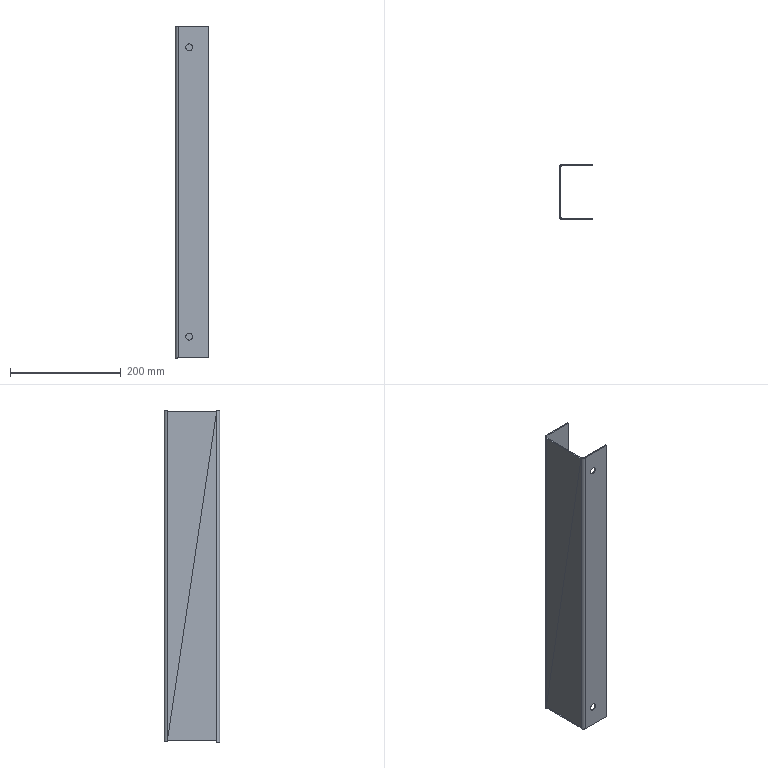Component | SolidWorks | Base-1_BaseLeft-Right-2 | 1 solid | 36 faces | box 60 x 100 x 600 mm | volume 252871 mm3 | plane 24 | cylinder 12 | commonest cylinder face diameters 12.5 x8 7 x2 11 x2
STEP:
#1=COLOUR_RGB('',0.7922,0.8196,0.9333);
#2=FILL_AREA_STYLE_COLOUR('',#1);
#3=FILL_AREA_STYLE('',(#2));
#4=SURFACE_STYLE_FILL_AREA(#3);
#5=SURFACE_SIDE_STYLE('',(#4));
#6=SURFACE_STYLE_USAGE(.BOTH.,#5);
#7=PRESENTATION_STYLE_ASSIGNMENT((#6));
#8=CARTESIAN_POINT('',(-17.788,-8.801,14.723));
#9=VERTEX_POINT('',#8);
#10=CARTESIAN_POINT('',(-18.28,-8.801,14.723));
#11=VERTEX_POINT('',#10);
#12=CARTESIAN_POINT('',(-18.034,-8.801,14.723));
#13=DIRECTION('',(0.,-1.,-0.));
#14=DIRECTION('',(1.,0.,0.));
#15=AXIS2_PLACEMENT_3D('',#12,#13,#14);
#16=CIRCLE('',#15,0.2461);
#17=EDGE_CURVE('',#9,#11,#16,.T.);
#18=ORIENTED_EDGE('',*,*,#17,.F.);
#19=CARTESIAN_POINT('',(-17.788,-8.88,14.723));
#20=VERTEX_POINT('',#19);
#21=CARTESIAN_POINT('',(-17.788,-4.942,14.723));
#22=DIRECTION('',(0.,-1.,-0.));
#23=VECTOR('',#22,39.37);
#24=LINE('',#21,#23);
#25=EDGE_CURVE('',#9,#20,#24,.T.);
#26=ORIENTED_EDGE('',*,*,#25,.T.);
#27=CARTESIAN_POINT('',(-18.28,-8.88,14.723));
#28=VERTEX_POINT('',#27);
#29=CARTESIAN_POINT('',(-18.034,-8.88,14.723));
#30=DIRECTION('',(0.,-1.,-0.));
#31=DIRECTION('',(-1.,-0.,-0.));
#32=AXIS2_PLACEMENT_3D('',#29,#30,#31);
#33=CIRCLE('',#32,0.2461);
#34=EDGE_CURVE('',#20,#28,#33,.T.);
#35=ORIENTED_EDGE('',*,*,#34,.T.);
#36=CARTESIAN_POINT('',(-18.28,-4.942,14.723));
#37=DIRECTION('',(0.,-1.,-0.));
#38=VECTOR('',#37,39.37);
#39=LINE('',#36,#38);
#40=EDGE_CURVE('',#11,#28,#39,.T.);
#41=ORIENTED_EDGE('',*,*,#40,.F.);
#42=EDGE_LOOP('',(#18,#26,#35,#41));
#43=FACE_OUTER_BOUND('',#42,.T.);
#44=CARTESIAN_POINT('',(-18.034,-4.942,14.723));
#45=DIRECTION('',(0.,-1.,-0.));
#46=DIRECTION('',(-1.,-0.,-0.));
#47=AXIS2_PLACEMENT_3D('',#44,#45,#46);
#48=CYLINDRICAL_SURFACE('',#47,0.2461);
#49=ADVANCED_FACE('',(#43),#48,.F.);
#50=CARTESIAN_POINT('',(-17.788,-8.801,-5.867));
#51=VERTEX_POINT('',#50);
#52=CARTESIAN_POINT('',(-18.28,-8.801,-5.867));
#53=VERTEX_POINT('',#52);
#54=CARTESIAN_POINT('',(-18.034,-8.801,-5.867));
#55=DIRECTION('',(0.,-1.,-0.));
#56=DIRECTION('',(1.,0.,0.));
#57=AXIS2_PLACEMENT_3D('',#54,#55,#56);
#58=CIRCLE('',#57,0.2461);
#59=EDGE_CURVE('',#51,#53,#58,.T.);
#60=ORIENTED_EDGE('',*,*,#59,.F.);
#61=CARTESIAN_POINT('',(-17.788,-8.88,-5.867));
#62=VERTEX_POINT('',#61);
#63=CARTESIAN_POINT('',(-17.788,-4.942,-5.867));
#64=DIRECTION('',(0.,-1.,-0.));
#65=VECTOR('',#64,39.37);
#66=LINE('',#63,#65);
#67=EDGE_CURVE('',#51,#62,#66,.T.);
#68=ORIENTED_EDGE('',*,*,#67,.T.);
#69=CARTESIAN_POINT('',(-18.28,-8.88,-5.867));
#70=VERTEX_POINT('',#69);
#71=CARTESIAN_POINT('',(-18.034,-8.88,-5.867));
#72=DIRECTION('',(0.,-1.,-0.));
#73=DIRECTION('',(-1.,-0.,-0.));
#74=AXIS2_PLACEMENT_3D('',#71,#72,#73);
#75=CIRCLE('',#74,0.2461);
#76=EDGE_CURVE('',#62,#70,#75,.T.);
#77=ORIENTED_EDGE('',*,*,#76,.T.);
#78=CARTESIAN_POINT('',(-18.28,-4.942,-5.867));
#79=DIRECTION('',(0.,-1.,-0.));
#80=VECTOR('',#79,39.37);
#81=LINE('',#78,#80);
#82=EDGE_CURVE('',#53,#70,#81,.T.);
#83=ORIENTED_EDGE('',*,*,#82,.F.);
#84=EDGE_LOOP('',(#60,#68,#77,#83));
#85=FACE_OUTER_BOUND('',#84,.T.);
#86=CARTESIAN_POINT('',(-18.034,-4.942,-5.867));
#87=DIRECTION('',(0.,-1.,-0.));
#88=DIRECTION('',(-1.,-0.,-0.));
#89=AXIS2_PLACEMENT_3D('',#86,#87,#88);
#90=CYLINDRICAL_SURFACE('',#89,0.2461);
#91=ADVANCED_FACE('',(#85),#90,.F.);
#92=CARTESIAN_POINT('',(-18.28,-5.021,12.105));
#93=VERTEX_POINT('',#92);
#94=CARTESIAN_POINT('',(-17.788,-5.021,12.105));
#95=VERTEX_POINT('',#94);
#96=CARTESIAN_POINT('',(-18.034,-5.021,12.105));
#97=DIRECTION('',(-0.,1.,0.));
#98=DIRECTION('',(-1.,-0.,-0.));
#99=AXIS2_PLACEMENT_3D('',#96,#97,#98);
#100=CIRCLE('',#99,0.2461);
#101=EDGE_CURVE('',#93,#95,#100,.T.);
#102=ORIENTED_EDGE('',*,*,#101,.F.);
#103=CARTESIAN_POINT('',(-18.28,-4.943,12.105));
#104=VERTEX_POINT('',#103);
#105=CARTESIAN_POINT('',(-18.28,-8.88,12.105));
#106=DIRECTION('',(-0.,1.,0.));
#107=VECTOR('',#106,39.37);
#108=LINE('',#105,#107);
#109=EDGE_CURVE('',#93,#104,#108,.T.);
#110=ORIENTED_EDGE('',*,*,#109,.T.);
#111=CARTESIAN_POINT('',(-17.788,-4.943,12.105));
#112=VERTEX_POINT('',#111);
#113=CARTESIAN_POINT('',(-18.034,-4.943,12.105));
#114=DIRECTION('',(-0.,1.,0.));
#115=DIRECTION('',(1.,0.,0.));
#116=AXIS2_PLACEMENT_3D('',#113,#114,#115);
#117=CIRCLE('',#116,0.2461);
#118=EDGE_CURVE('',#104,#112,#117,.T.);
#119=ORIENTED_EDGE('',*,*,#118,.T.);
#120=CARTESIAN_POINT('',(-17.788,-8.88,12.105));
#121=DIRECTION('',(-0.,1.,0.));
#122=VECTOR('',#121,39.37);
#123=LINE('',#120,#122);
#124=EDGE_CURVE('',#95,#112,#123,.T.);
#125=ORIENTED_EDGE('',*,*,#124,.F.);
#126=EDGE_LOOP('',(#102,#110,#119,#125));
#127=FACE_OUTER_BOUND('',#126,.T.);
#128=CARTESIAN_POINT('',(-18.034,-8.88,12.105));
#129=DIRECTION('',(-0.,1.,0.));
#130=DIRECTION('',(1.,0.,0.));
#131=AXIS2_PLACEMENT_3D('',#128,#129,#130);
#132=CYLINDRICAL_SURFACE('',#131,0.2461);
#133=ADVANCED_FACE('',(#127),#132,.F.);
#134=CARTESIAN_POINT('',(-18.28,-5.021,-3.249));
#135=VERTEX_POINT('',#134);
#136=CARTESIAN_POINT('',(-17.788,-5.021,-3.249));
#137=VERTEX_POINT('',#136);
#138=CARTESIAN_POINT('',(-18.034,-5.021,-3.249));
#139=DIRECTION('',(-0.,1.,0.));
#140=DIRECTION('',(-1.,-0.,-0.));
#141=AXIS2_PLACEMENT_3D('',#138,#139,#140);
#142=CIRCLE('',#141,0.2461);
#143=EDGE_CURVE('',#135,#137,#142,.T.);
#144=ORIENTED_EDGE('',*,*,#143,.F.);
#145=CARTESIAN_POINT('',(-18.28,-4.943,-3.249));
#146=VERTEX_POINT('',#145);
#147=CARTESIAN_POINT('',(-18.28,-8.88,-3.249));
#148=DIRECTION('',(-0.,1.,0.));
#149=VECTOR('',#148,39.37);
#150=LINE('',#147,#149);
#151=EDGE_CURVE('',#135,#146,#150,.T.);
#152=ORIENTED_EDGE('',*,*,#151,.T.);
#153=CARTESIAN_POINT('',(-17.788,-4.943,-3.249));
#154=VERTEX_POINT('',#153);
#155=CARTESIAN_POINT('',(-18.034,-4.943,-3.249));
#156=DIRECTION('',(-0.,1.,0.));
#157=DIRECTION('',(1.,0.,0.));
#158=AXIS2_PLACEMENT_3D('',#155,#156,#157);
#159=CIRCLE('',#158,0.2461);
#160=EDGE_CURVE('',#146,#154,#159,.T.);
#161=ORIENTED_EDGE('',*,*,#160,.T.);
#162=CARTESIAN_POINT('',(-17.788,-8.88,-3.249));
#163=DIRECTION('',(-0.,1.,0.));
#164=VECTOR('',#163,39.37);
#165=LINE('',#162,#164);
#166=EDGE_CURVE('',#137,#154,#165,.T.);
#167=ORIENTED_EDGE('',*,*,#166,.F.);
#168=EDGE_LOOP('',(#144,#152,#161,#167));
#169=FACE_OUTER_BOUND('',#168,.T.);
#170=CARTESIAN_POINT('',(-18.034,-8.88,-3.249));
#171=DIRECTION('',(-0.,1.,0.));
#172=DIRECTION('',(1.,0.,0.));
#173=AXIS2_PLACEMENT_3D('',#170,#171,#172);
#174=CYLINDRICAL_SURFACE('',#173,0.2461);
#175=ADVANCED_FACE('',(#169),#174,.F.);
#176=CARTESIAN_POINT('',(-18.939,-8.663,16.239));
#177=VERTEX_POINT('',#176);
#178=CARTESIAN_POINT('',(-18.939,-8.663,16.239));
#179=VERTEX_POINT('',#178);
#180=CARTESIAN_POINT('',(-18.939,-8.88,16.239));
#181=DIRECTION('',(-0.,1.,0.));
#182=VECTOR('',#181,39.37);
#183=LINE('',#180,#182);
#184=EDGE_CURVE('',#177,#179,#183,.T.);
#185=ORIENTED_EDGE('',*,*,#184,.T.);
#186=CARTESIAN_POINT('',(-19.018,-8.663,16.239));
#187=VERTEX_POINT('',#186);
#188=CARTESIAN_POINT('',(-18.802,-8.663,16.239));
#189=DIRECTION('',(-1.,-0.,-0.));
#190=VECTOR('',#189,39.37);
#191=LINE('',#188,#190);
#192=EDGE_CURVE('',#179,#187,#191,.T.);
#193=ORIENTED_EDGE('',*,*,#192,.T.);
#194=CARTESIAN_POINT('',(-19.018,-8.663,16.239));
#195=DIRECTION('',(1.,0.,0.));
#196=VECTOR('',#195,39.37);
#197=LINE('',#194,#196);
#198=EDGE_CURVE('',#187,#177,#197,.T.);
#199=ORIENTED_EDGE('',*,*,#198,.T.);
#200=EDGE_LOOP('',(#185,#193,#199));
#201=FACE_OUTER_BOUND('',#200,.T.);
#202=CARTESIAN_POINT('',(-18.802,-8.801,16.239));
#203=DIRECTION('',(-0.,-0.,1.));
#204=DIRECTION('',(1.,0.,0.));
#205=AXIS2_PLACEMENT_3D('',#202,#203,#204);
#206=PLANE('',#205);
#207=ADVANCED_FACE('',(#201),#206,.T.);
#208=CARTESIAN_POINT('',(-18.939,-5.159,-7.383));
#209=VERTEX_POINT('',#208);
#210=CARTESIAN_POINT('',(-18.802,-5.021,-7.383));
#211=VERTEX_POINT('',#210);
#212=CARTESIAN_POINT('',(-18.802,-5.159,-7.383));
#213=DIRECTION('',(0.,0.,-1.));
#214=DIRECTION('',(-0.,1.,0.));
#215=AXIS2_PLACEMENT_3D('',#212,#213,#214);
#216=CIRCLE('',#215,0.1378);
#217=EDGE_CURVE('',#209,#211,#216,.T.);
#218=ORIENTED_EDGE('',*,*,#217,.F.);
#219=CARTESIAN_POINT('',(-19.018,-5.159,-7.383));
#220=VERTEX_POINT('',#219);
#221=CARTESIAN_POINT('',(-19.018,-5.159,-7.383));
#222=DIRECTION('',(-1.,-0.,-0.));
#223=VECTOR('',#222,39.37);
#224=LINE('',#221,#223);
#225=EDGE_CURVE('',#209,#220,#224,.T.);
#226=ORIENTED_EDGE('',*,*,#225,.T.);
#227=CARTESIAN_POINT('',(-18.802,-4.943,-7.383));
#228=VERTEX_POINT('',#227);
#229=CARTESIAN_POINT('',(-18.802,-5.159,-7.383));
#230=DIRECTION('',(0.,0.,-1.));
#231=DIRECTION('',(1.,0.,0.));
#232=AXIS2_PLACEMENT_3D('',#229,#230,#231);
#233=CIRCLE('',#232,0.2165);
#234=EDGE_CURVE('',#220,#228,#233,.T.);
#235=ORIENTED_EDGE('',*,*,#234,.T.);
#236=CARTESIAN_POINT('',(-18.802,-5.021,-7.383));
#237=DIRECTION('',(-0.,1.,0.));
#238=VECTOR('',#237,39.37);
#239=LINE('',#236,#238);
#240=EDGE_CURVE('',#211,#228,#239,.T.);
#241=ORIENTED_EDGE('',*,*,#240,.F.);
#242=EDGE_LOOP('',(#218,#226,#235,#241));
#243=FACE_OUTER_BOUND('',#242,.T.);
#244=CARTESIAN_POINT('',(-19.018,-5.159,-7.383));
#245=DIRECTION('',(0.,0.,-1.));
#246=DIRECTION('',(-1.,-0.,-0.));
#247=AXIS2_PLACEMENT_3D('',#244,#245,#246);
#248=PLANE('',#247);
#249=ADVANCED_FACE('',(#243),#248,.T.);
#250=CARTESIAN_POINT('',(-18.939,-8.663,-7.383));
#251=VERTEX_POINT('',#250);
#252=CARTESIAN_POINT('',(-19.018,-8.663,-7.383));
#253=VERTEX_POINT('',#252);
#254=CARTESIAN_POINT('',(-18.939,-8.663,-7.383));
#255=DIRECTION('',(-1.,-0.,-0.));
#256=VECTOR('',#255,39.37);
#257=LINE('',#254,#256);
#258=EDGE_CURVE('',#251,#253,#257,.T.);
#259=ORIENTED_EDGE('',*,*,#258,.T.);
#260=CARTESIAN_POINT('',(-18.939,-8.663,-7.383));
#261=VERTEX_POINT('',#260);
#262=CARTESIAN_POINT('',(-18.802,-8.663,-7.383));
#263=DIRECTION('',(1.,0.,0.));
#264=VECTOR('',#263,39.37);
#265=LINE('',#262,#264);
#266=EDGE_CURVE('',#253,#261,#265,.T.);
#267=ORIENTED_EDGE('',*,*,#266,.T.);
#268=CARTESIAN_POINT('',(-18.939,-8.88,-7.383));
#269=DIRECTION('',(-0.,1.,0.));
#270=VECTOR('',#269,39.37);
#271=LINE('',#268,#270);
#272=EDGE_CURVE('',#251,#261,#271,.T.);
#273=ORIENTED_EDGE('',*,*,#272,.F.);
#274=EDGE_LOOP('',(#259,#267,#273));
#275=FACE_OUTER_BOUND('',#274,.T.);
#276=CARTESIAN_POINT('',(-18.802,-5.021,-7.383));
#277=DIRECTION('',(0.,0.,-1.));
#278=DIRECTION('',(-1.,-0.,-0.));
#279=AXIS2_PLACEMENT_3D('',#276,#277,#278);
#280=PLANE('',#279);
#281=ADVANCED_FACE('',(#275),#280,.T.);
#282=CARTESIAN_POINT('',(-19.018,-5.159,16.239));
#283=VERTEX_POINT('',#282);
#284=CARTESIAN_POINT('',(-18.802,-4.943,16.239));
#285=VERTEX_POINT('',#284);
#286=CARTESIAN_POINT('',(-18.802,-5.159,16.239));
#287=DIRECTION('',(0.,0.,-1.));
#288=DIRECTION('',(1.,0.,0.));
#289=AXIS2_PLACEMENT_3D('',#286,#287,#288);
#290=CIRCLE('',#289,0.2165);
#291=EDGE_CURVE('',#283,#285,#290,.T.);
#292=ORIENTED_EDGE('',*,*,#291,.F.);
#293=CARTESIAN_POINT('',(-18.939,-5.159,16.239));
#294=VERTEX_POINT('',#293);
#295=CARTESIAN_POINT('',(-18.802,-5.159,16.239));
#296=DIRECTION('',(1.,0.,0.));
#297=VECTOR('',#296,39.37);
#298=LINE('',#295,#297);
#299=EDGE_CURVE('',#283,#294,#298,.T.);
#300=ORIENTED_EDGE('',*,*,#299,.T.);
#301=CARTESIAN_POINT('',(-18.802,-5.021,16.239));
#302=VERTEX_POINT('',#301);
#303=CARTESIAN_POINT('',(-18.802,-5.159,16.239));
#304=DIRECTION('',(0.,0.,-1.));
#305=DIRECTION('',(-0.,1.,0.));
#306=AXIS2_PLACEMENT_3D('',#303,#304,#305);
#307=CIRCLE('',#306,0.1378);
#308=EDGE_CURVE('',#294,#302,#307,.T.);
#309=ORIENTED_EDGE('',*,*,#308,.T.);
#310=CARTESIAN_POINT('',(-18.802,-4.943,16.239));
#311=DIRECTION('',(0.,-1.,-0.));
#312=VECTOR('',#311,39.37);
#313=LINE('',#310,#312);
#314=EDGE_CURVE('',#285,#302,#313,.T.);
#315=ORIENTED_EDGE('',*,*,#314,.F.);
#316=EDGE_LOOP('',(#292,#300,#309,#315));
#317=FACE_OUTER_BOUND('',#316,.T.);
#318=CARTESIAN_POINT('',(-18.802,-4.943,16.239));
#319=DIRECTION('',(-0.,-0.,1.));
#320=DIRECTION('',(1.,0.,0.));
#321=AXIS2_PLACEMENT_3D('',#318,#319,#320);
#322=PLANE('',#321);
#323=ADVANCED_FACE('',(#317),#322,.T.);
#324=ORIENTED_EDGE('',*,*,#308,.F.);
#325=CARTESIAN_POINT('',(-18.939,-5.159,16.16));
#326=VERTEX_POINT('',#325);
#327=CARTESIAN_POINT('',(-18.939,-5.159,-7.383));
#328=DIRECTION('',(0.,0.,-1.));
#329=VECTOR('',#328,39.37);
#330=LINE('',#327,#329);
#331=EDGE_CURVE('',#294,#326,#330,.T.);
#332=ORIENTED_EDGE('',*,*,#331,.T.);
#333=CARTESIAN_POINT('',(-18.939,-5.159,-7.304));
#334=VERTEX_POINT('',#333);
#335=CARTESIAN_POINT('',(-18.939,-5.159,-7.383));
#336=DIRECTION('',(-0.,-0.,1.));
#337=VECTOR('',#336,39.37);
#338=LINE('',#335,#337);
#339=EDGE_CURVE('',#334,#326,#338,.T.);
#340=ORIENTED_EDGE('',*,*,#339,.F.);
#341=CARTESIAN_POINT('',(-18.939,-5.159,-7.383));
#342=DIRECTION('',(0.,0.,-1.));
#343=VECTOR('',#342,39.37);
#344=LINE('',#341,#343);
#345=EDGE_CURVE('',#334,#209,#344,.T.);
#346=ORIENTED_EDGE('',*,*,#345,.T.);
#347=ORIENTED_EDGE('',*,*,#217,.T.);
#348=CARTESIAN_POINT('',(-18.802,-5.021,-7.383));
#349=DIRECTION('',(-0.,-0.,1.));
#350=VECTOR('',#349,39.37);
#351=LINE('',#348,#350);
#352=EDGE_CURVE('',#211,#302,#351,.T.);
#353=ORIENTED_EDGE('',*,*,#352,.T.);
#354=EDGE_LOOP('',(#324,#332,#340,#346,#347,#353));
#355=FACE_OUTER_BOUND('',#354,.T.);
#356=CARTESIAN_POINT('',(-18.802,-5.159,-7.383));
#357=DIRECTION('',(-0.,-0.,1.));
#358=DIRECTION('',(1.,0.,0.));
#359=AXIS2_PLACEMENT_3D('',#356,#357,#358);
#360=CYLINDRICAL_SURFACE('',#359,0.1378);
#361=ADVANCED_FACE('',(#355),#360,.F.);
#362=CARTESIAN_POINT('',(-18.939,-8.663,16.16));
#363=VERTEX_POINT('',#362);
#364=CARTESIAN_POINT('',(-18.939,-8.88,16.16));
#365=DIRECTION('',(0.,-1.,-0.));
#366=VECTOR('',#365,39.37);
#367=LINE('',#364,#366);
#368=EDGE_CURVE('',#326,#363,#367,.T.);
#369=ORIENTED_EDGE('',*,*,#368,.T.);
#370=CARTESIAN_POINT('',(-18.939,-8.663,-7.383));
#371=DIRECTION('',(-0.,-0.,1.));
#372=VECTOR('',#371,39.37);
#373=LINE('',#370,#372);
#374=EDGE_CURVE('',#363,#179,#373,.T.);
#375=ORIENTED_EDGE('',*,*,#374,.T.);
#376=ORIENTED_EDGE('',*,*,#184,.F.);
#377=CARTESIAN_POINT('',(-18.939,-8.663,-7.383));
#378=DIRECTION('',(-0.,-0.,1.));
#379=VECTOR('',#378,39.37);
#380=LINE('',#377,#379);
#381=EDGE_CURVE('',#251,#177,#380,.T.);
#382=ORIENTED_EDGE('',*,*,#381,.F.);
#383=ORIENTED_EDGE('',*,*,#272,.T.);
#384=CARTESIAN_POINT('',(-18.939,-8.663,-7.304));
#385=VERTEX_POINT('',#384);
#386=CARTESIAN_POINT('',(-18.939,-8.663,-7.383));
#387=DIRECTION('',(-0.,-0.,1.));
#388=VECTOR('',#387,39.37);
#389=LINE('',#386,#388);
#390=EDGE_CURVE('',#261,#385,#389,.T.);
#391=ORIENTED_EDGE('',*,*,#390,.T.);
#392=CARTESIAN_POINT('',(-18.939,-8.88,-7.304));
#393=DIRECTION('',(-0.,1.,0.));
#394=VECTOR('',#393,39.37);
#395=LINE('',#392,#394);
#396=EDGE_CURVE('',#385,#334,#395,.T.);
#397=ORIENTED_EDGE('',*,*,#396,.T.);
#398=ORIENTED_EDGE('',*,*,#339,.T.);
#399=EDGE_LOOP('',(#369,#375,#376,#382,#383,#391,#397,#398));
#400=FACE_OUTER_BOUND('',#399,.T.);
#401=CARTESIAN_POINT('',(-18.939,-8.88,-7.383));
#402=DIRECTION('',(1.,0.,0.));
#403=DIRECTION('',(0.,-1.,-0.));
#404=AXIS2_PLACEMENT_3D('',#401,#402,#403);
#405=PLANE('',#404);
#406=ADVANCED_FACE('',(#400),#405,.T.);
#407=CARTESIAN_POINT('',(-19.018,-8.663,16.16));
#408=VERTEX_POINT('',#407);
#409=CARTESIAN_POINT('',(-19.018,-8.663,16.259));
#410=DIRECTION('',(-0.,-0.,1.));
#411=VECTOR('',#410,39.37);
#412=LINE('',#409,#411);
#413=EDGE_CURVE('',#408,#187,#412,.T.);
#414=ORIENTED_EDGE('',*,*,#413,.F.);
#415=CARTESIAN_POINT('',(-19.018,-5.159,16.16));
#416=VERTEX_POINT('',#415);
#417=CARTESIAN_POINT('',(-19.018,-8.663,16.16));
#418=DIRECTION('',(0.,-1.,-0.));
#419=VECTOR('',#418,39.37);
#420=LINE('',#417,#419);
#421=EDGE_CURVE('',#416,#408,#420,.T.);
#422=ORIENTED_EDGE('',*,*,#421,.F.);
#423=CARTESIAN_POINT('',(-19.018,-5.159,-7.304));
#424=VERTEX_POINT('',#423);
#425=CARTESIAN_POINT('',(-19.018,-5.159,-7.383));
#426=DIRECTION('',(-0.,-0.,1.));
#427=VECTOR('',#426,39.37);
#428=LINE('',#425,#427);
#429=EDGE_CURVE('',#424,#416,#428,.T.);
#430=ORIENTED_EDGE('',*,*,#429,.F.);
#431=CARTESIAN_POINT('',(-19.018,-8.663,-7.304));
#432=VERTEX_POINT('',#431);
#433=CARTESIAN_POINT('',(-19.018,-8.663,-7.304));
#434=DIRECTION('',(-0.,1.,0.));
#435=VECTOR('',#434,39.37);
#436=LINE('',#433,#435);
#437=EDGE_CURVE('',#432,#424,#436,.T.);
#438=ORIENTED_EDGE('',*,*,#437,.F.);
#439=CARTESIAN_POINT('',(-19.018,-8.663,-7.304));
#440=DIRECTION('',(-0.,-0.,1.));
#441=VECTOR('',#440,39.37);
#442=LINE('',#439,#441);
#443=EDGE_CURVE('',#253,#432,#442,.T.);
#444=ORIENTED_EDGE('',*,*,#443,.F.);
#445=CARTESIAN_POINT('',(-19.018,-8.663,-7.383));
#446=DIRECTION('',(-0.,-0.,1.));
#447=VECTOR('',#446,39.37);
#448=LINE('',#445,#447);
#449=EDGE_CURVE('',#253,#187,#448,.T.);
#450=ORIENTED_EDGE('',*,*,#449,.T.);
#451=EDGE_LOOP('',(#414,#422,#430,#438,#444,#450));
#452=FACE_OUTER_BOUND('',#451,.T.);
#453=CARTESIAN_POINT('',(-19.018,-8.88,-7.383));
#454=DIRECTION('',(1.,0.,0.));
#455=DIRECTION('',(0.,-1.,-0.));
#456=AXIS2_PLACEMENT_3D('',#453,#454,#455);
#457=PLANE('',#456);
#458=ADVANCED_FACE('',(#452),#457,.F.);
#459=CARTESIAN_POINT('',(-18.802,-8.88,-7.383));
#460=VERTEX_POINT('',#459);
#461=CARTESIAN_POINT('',(-18.802,-8.801,-7.383));
#462=VERTEX_POINT('',#461);
#463=CARTESIAN_POINT('',(-18.802,-8.88,-7.383));
#464=DIRECTION('',(-0.,1.,0.));
#465=VECTOR('',#464,39.37);
#466=LINE('',#463,#465);
#467=EDGE_CURVE('',#460,#462,#466,.T.);
#468=ORIENTED_EDGE('',*,*,#467,.F.);
#469=CARTESIAN_POINT('',(-18.802,-8.663,-7.383));
#470=DIRECTION('',(0.,0.,-1.));
#471=DIRECTION('',(1.,0.,0.));
#472=AXIS2_PLACEMENT_3D('',#469,#470,#471);
#473=CIRCLE('',#472,0.2165);
#474=EDGE_CURVE('',#460,#253,#473,.T.);
#475=ORIENTED_EDGE('',*,*,#474,.T.);
#476=ORIENTED_EDGE('',*,*,#258,.F.);
#477=CARTESIAN_POINT('',(-18.802,-8.663,-7.383));
#478=DIRECTION('',(0.,0.,-1.));
#479=DIRECTION('',(-0.,1.,0.));
#480=AXIS2_PLACEMENT_3D('',#477,#478,#479);
#481=CIRCLE('',#480,0.1378);
#482=EDGE_CURVE('',#462,#251,#481,.T.);
#483=ORIENTED_EDGE('',*,*,#482,.F.);
#484=EDGE_LOOP('',(#468,#475,#476,#483));
#485=FACE_OUTER_BOUND('',#484,.T.);
#486=CARTESIAN_POINT('',(-18.802,-8.88,-7.383));
#487=DIRECTION('',(0.,0.,-1.));
#488=DIRECTION('',(-1.,-0.,-0.));
#489=AXIS2_PLACEMENT_3D('',#486,#487,#488);
#490=PLANE('',#489);
#491=ADVANCED_FACE('',(#485),#490,.T.);
#492=CARTESIAN_POINT('',(-16.656,-8.88,-7.383));
#493=VERTEX_POINT('',#492);
#494=CARTESIAN_POINT('',(-16.656,-8.88,-7.383));
#495=DIRECTION('',(-1.,-0.,-0.));
#496=VECTOR('',#495,39.37);
#497=LINE('',#494,#496);
#498=EDGE_CURVE('',#493,#460,#497,.T.);
#499=ORIENTED_EDGE('',*,*,#498,.T.);
#500=ORIENTED_EDGE('',*,*,#467,.T.);
#501=CARTESIAN_POINT('',(-16.656,-8.801,-7.383));
#502=VERTEX_POINT('',#501);
#503=CARTESIAN_POINT('',(-16.656,-8.801,-7.383));
#504=DIRECTION('',(-1.,-0.,-0.));
#505=VECTOR('',#504,39.37);
#506=LINE('',#503,#505);
#507=EDGE_CURVE('',#502,#462,#506,.T.);
#508=ORIENTED_EDGE('',*,*,#507,.F.);
#509=CARTESIAN_POINT('',(-16.656,-8.88,-7.383));
#510=DIRECTION('',(-0.,1.,0.));
#511=VECTOR('',#510,39.37);
#512=LINE('',#509,#511);
#513=EDGE_CURVE('',#493,#502,#512,.T.);
#514=ORIENTED_EDGE('',*,*,#513,.F.);
#515=EDGE_LOOP('',(#499,#500,#508,#514));
#516=FACE_OUTER_BOUND('',#515,.T.);
#517=CARTESIAN_POINT('',(-18.939,-8.663,-7.383));
#518=DIRECTION('',(0.,0.,-1.));
#519=DIRECTION('',(-1.,-0.,-0.));
#520=AXIS2_PLACEMENT_3D('',#517,#518,#519);
#521=PLANE('',#520);
#522=ADVANCED_FACE('',(#516),#521,.T.);
#523=ORIENTED_EDGE('',*,*,#198,.F.);
#524=CARTESIAN_POINT('',(-18.802,-8.88,16.239));
#525=VERTEX_POINT('',#524);
#526=CARTESIAN_POINT('',(-18.802,-8.663,16.239));
#527=DIRECTION('',(0.,0.,-1.));
#528=DIRECTION('',(1.,0.,0.));
#529=AXIS2_PLACEMENT_3D('',#526,#527,#528);
#530=CIRCLE('',#529,0.2165);
#531=EDGE_CURVE('',#525,#187,#530,.T.);
#532=ORIENTED_EDGE('',*,*,#531,.F.);
#533=CARTESIAN_POINT('',(-18.802,-8.801,16.239));
#534=VERTEX_POINT('',#533);
#535=CARTESIAN_POINT('',(-18.802,-8.801,16.239));
#536=DIRECTION('',(0.,-1.,-0.));
#537=VECTOR('',#536,39.37);
#538=LINE('',#535,#537);
#539=EDGE_CURVE('',#534,#525,#538,.T.);
#540=ORIENTED_EDGE('',*,*,#539,.F.);
#541=CARTESIAN_POINT('',(-18.802,-8.663,16.239));
#542=DIRECTION('',(0.,0.,-1.));
#543=DIRECTION('',(-0.,1.,0.));
#544=AXIS2_PLACEMENT_3D('',#541,#542,#543);
#545=CIRCLE('',#544,0.1378);
#546=EDGE_CURVE('',#534,#177,#545,.T.);
#547=ORIENTED_EDGE('',*,*,#546,.T.);
#548=EDGE_LOOP('',(#523,#532,#540,#547));
#549=FACE_OUTER_BOUND('',#548,.T.);
#550=CARTESIAN_POINT('',(-19.018,-8.663,16.239));
#551=DIRECTION('',(-0.,-0.,1.));
#552=DIRECTION('',(1.,0.,0.));
#553=AXIS2_PLACEMENT_3D('',#550,#551,#552);
#554=PLANE('',#553);
#555=ADVANCED_FACE('',(#549),#554,.T.);
#556=CARTESIAN_POINT('',(-16.656,-4.943,16.239));
#557=VERTEX_POINT('',#556);
#558=CARTESIAN_POINT('',(-19.018,-4.943,16.239));
#559=DIRECTION('',(1.,0.,0.));
#560=VECTOR('',#559,39.37);
#561=LINE('',#558,#560);
#562=EDGE_CURVE('',#285,#557,#561,.T.);
#563=ORIENTED_EDGE('',*,*,#562,.F.);
#564=ORIENTED_EDGE('',*,*,#314,.T.);
#565=CARTESIAN_POINT('',(-16.656,-5.021,16.239));
#566=VERTEX_POINT('',#565);
#567=CARTESIAN_POINT('',(-19.018,-5.021,16.239));
#568=DIRECTION('',(1.,0.,0.));
#569=VECTOR('',#568,39.37);
#570=LINE('',#567,#569);
#571=EDGE_CURVE('',#302,#566,#570,.T.);
#572=ORIENTED_EDGE('',*,*,#571,.T.);
#573=CARTESIAN_POINT('',(-16.656,-5.021,16.239));
#574=DIRECTION('',(-0.,1.,0.));
#575=VECTOR('',#574,39.37);
#576=LINE('',#573,#575);
#577=EDGE_CURVE('',#566,#557,#576,.T.);
#578=ORIENTED_EDGE('',*,*,#577,.T.);
#579=EDGE_LOOP('',(#563,#564,#572,#578));
#580=FACE_OUTER_BOUND('',#579,.T.);
#581=CARTESIAN_POINT('',(-18.939,-5.159,16.239));
#582=DIRECTION('',(-0.,-0.,1.));
#583=DIRECTION('',(1.,0.,0.));
#584=AXIS2_PLACEMENT_3D('',#581,#582,#583);
#585=PLANE('',#584);
#586=ADVANCED_FACE('',(#580),#585,.T.);
#587=CARTESIAN_POINT('',(-18.034,-4.943,12.105));
#588=DIRECTION('',(-0.,1.,0.));
#589=DIRECTION('',(1.,0.,0.));
#590=AXIS2_PLACEMENT_3D('',#587,#588,#589);
#591=CIRCLE('',#590,0.2461);
#592=EDGE_CURVE('',#112,#104,#591,.T.);
#593=ORIENTED_EDGE('',*,*,#592,.F.);
#594=ORIENTED_EDGE('',*,*,#118,.F.);
#595=EDGE_LOOP('',(#593,#594));
#596=FACE_BOUND('',#595,.T.);
#597=CARTESIAN_POINT('',(-18.034,-4.943,-3.249));
#598=DIRECTION('',(-0.,1.,0.));
#599=DIRECTION('',(1.,0.,0.));
#600=AXIS2_PLACEMENT_3D('',#597,#598,#599);
#601=CIRCLE('',#600,0.2461);
#602=EDGE_CURVE('',#154,#146,#601,.T.);
#603=ORIENTED_EDGE('',*,*,#602,.F.);
#604=ORIENTED_EDGE('',*,*,#160,.F.);
#605=EDGE_LOOP('',(#603,#604));
#606=FACE_BOUND('',#605,.T.);
#607=ORIENTED_EDGE('',*,*,#562,.T.);
#608=CARTESIAN_POINT('',(-16.656,-4.943,-7.383));
#609=VERTEX_POINT('',#608);
#610=CARTESIAN_POINT('',(-16.656,-4.943,-7.383));
#611=DIRECTION('',(-0.,-0.,1.));
#612=VECTOR('',#611,39.37);
#613=LINE('',#610,#612);
#614=EDGE_CURVE('',#609,#557,#613,.T.);
#615=ORIENTED_EDGE('',*,*,#614,.F.);
#616=CARTESIAN_POINT('',(-19.018,-4.943,-7.383));
#617=DIRECTION('',(1.,0.,0.));
#618=VECTOR('',#617,39.37);
#619=LINE('',#616,#618);
#620=EDGE_CURVE('',#228,#609,#619,.T.);
#621=ORIENTED_EDGE('',*,*,#620,.F.);
#622=CARTESIAN_POINT('',(-18.802,-4.943,-7.383));
#623=DIRECTION('',(-0.,-0.,1.));
#624=VECTOR('',#623,39.37);
#625=LINE('',#622,#624);
#626=EDGE_CURVE('',#228,#285,#625,.T.);
#627=ORIENTED_EDGE('',*,*,#626,.T.);
#628=EDGE_LOOP('',(#607,#615,#621,#627));
#629=FACE_OUTER_BOUND('',#628,.T.);
#630=CARTESIAN_POINT('',(-19.018,-4.943,-7.383));
#631=DIRECTION('',(0.,-1.,-0.));
#632=DIRECTION('',(-1.,-0.,-0.));
#633=AXIS2_PLACEMENT_3D('',#630,#631,#632);
#634=PLANE('',#633);
#635=ADVANCED_FACE('',(#596,#606,#629),#634,.F.);
#636=ORIENTED_EDGE('',*,*,#577,.F.);
#637=CARTESIAN_POINT('',(-16.656,-5.021,-7.383));
#638=VERTEX_POINT('',#637);
#639=CARTESIAN_POINT('',(-16.656,-5.021,-7.383));
#640=DIRECTION('',(-0.,-0.,1.));
#641=VECTOR('',#640,39.37);
#642=LINE('',#639,#641);
#643=EDGE_CURVE('',#638,#566,#642,.T.);
#644=ORIENTED_EDGE('',*,*,#643,.F.);
#645=CARTESIAN_POINT('',(-16.656,-5.021,-7.383));
#646=DIRECTION('',(-0.,1.,0.));
#647=VECTOR('',#646,39.37);
#648=LINE('',#645,#647);
#649=EDGE_CURVE('',#638,#609,#648,.T.);
#650=ORIENTED_EDGE('',*,*,#649,.T.);
#651=ORIENTED_EDGE('',*,*,#614,.T.);
#652=EDGE_LOOP('',(#636,#644,#650,#651));
#653=FACE_OUTER_BOUND('',#652,.T.);
#654=CARTESIAN_POINT('',(-16.656,-5.021,-7.383));
#655=DIRECTION('',(1.,0.,0.));
#656=DIRECTION('',(0.,-1.,-0.));
#657=AXIS2_PLACEMENT_3D('',#654,#655,#656);
#658=PLANE('',#657);
#659=ADVANCED_FACE('',(#653),#658,.T.);
#660=CARTESIAN_POINT('',(-18.034,-5.021,12.105));
#661=DIRECTION('',(-0.,1.,0.));
#662=DIRECTION('',(-1.,-0.,-0.));
#663=AXIS2_PLACEMENT_3D('',#660,#661,#662);
#664=CIRCLE('',#663,0.2461);
#665=EDGE_CURVE('',#95,#93,#664,.T.);
#666=ORIENTED_EDGE('',*,*,#665,.T.);
#667=ORIENTED_EDGE('',*,*,#101,.T.);
#668=EDGE_LOOP('',(#666,#667));
#669=FACE_BOUND('',#668,.T.);
#670=CARTESIAN_POINT('',(-18.034,-5.021,-3.249));
#671=DIRECTION('',(-0.,1.,0.));
#672=DIRECTION('',(-1.,-0.,-0.));
#673=AXIS2_PLACEMENT_3D('',#670,#671,#672);
#674=CIRCLE('',#673,0.2461);
#675=EDGE_CURVE('',#137,#135,#674,.T.);
#676=ORIENTED_EDGE('',*,*,#675,.T.);
#677=ORIENTED_EDGE('',*,*,#143,.T.);
#678=EDGE_LOOP('',(#676,#677));
#679=FACE_BOUND('',#678,.T.);
#680=ORIENTED_EDGE('',*,*,#571,.F.);
#681=ORIENTED_EDGE('',*,*,#352,.F.);
#682=CARTESIAN_POINT('',(-19.018,-5.021,-7.383));
#683=DIRECTION('',(1.,0.,0.));
#684=VECTOR('',#683,39.37);
#685=LINE('',#682,#684);
#686=EDGE_CURVE('',#211,#638,#685,.T.);
#687=ORIENTED_EDGE('',*,*,#686,.T.);
#688=ORIENTED_EDGE('',*,*,#643,.T.);
#689=EDGE_LOOP('',(#680,#681,#687,#688));
#690=FACE_OUTER_BOUND('',#689,.T.);
#691=CARTESIAN_POINT('',(-19.018,-5.021,-7.383));
#692=DIRECTION('',(0.,-1.,-0.));
#693=DIRECTION('',(-1.,-0.,-0.));
#694=AXIS2_PLACEMENT_3D('',#691,#692,#693);
#695=PLANE('',#694);
#696=ADVANCED_FACE('',(#669,#679,#690),#695,.T.);
#697=ORIENTED_EDGE('',*,*,#546,.F.);
#698=CARTESIAN_POINT('',(-18.802,-8.801,-7.383));
#699=DIRECTION('',(-0.,-0.,1.));
#700=VECTOR('',#699,39.37);
#701=LINE('',#698,#700);
#702=EDGE_CURVE('',#462,#534,#701,.T.);
#703=ORIENTED_EDGE('',*,*,#702,.F.);
#704=ORIENTED_EDGE('',*,*,#482,.T.);
#705=ORIENTED_EDGE('',*,*,#381,.T.);
#706=EDGE_LOOP('',(#697,#703,#704,#705));
#707=FACE_OUTER_BOUND('',#706,.T.);
#708=CARTESIAN_POINT('',(-18.802,-8.663,-7.383));
#709=DIRECTION('',(-0.,-0.,1.));
#710=DIRECTION('',(1.,0.,0.));
#711=AXIS2_PLACEMENT_3D('',#708,#709,#710);
#712=CYLINDRICAL_SURFACE('',#711,0.1378);
#713=ADVANCED_FACE('',(#707),#712,.F.);
#714=CARTESIAN_POINT('',(-18.034,-8.801,14.723));
#715=DIRECTION('',(0.,-1.,-0.));
#716=DIRECTION('',(1.,0.,0.));
#717=AXIS2_PLACEMENT_3D('',#714,#715,#716);
#718=CIRCLE('',#717,0.2461);
#719=EDGE_CURVE('',#11,#9,#718,.T.);
#720=ORIENTED_EDGE('',*,*,#719,.T.);
#721=ORIENTED_EDGE('',*,*,#17,.T.);
#722=EDGE_LOOP('',(#720,#721));
#723=FACE_BOUND('',#722,.T.);
#724=CARTESIAN_POINT('',(-18.034,-8.801,-5.867));
#725=DIRECTION('',(0.,-1.,-0.));
#726=DIRECTION('',(1.,0.,0.));
#727=AXIS2_PLACEMENT_3D('',#724,#725,#726);
#728=CIRCLE('',#727,0.2461);
#729=EDGE_CURVE('',#53,#51,#728,.T.);
#730=ORIENTED_EDGE('',*,*,#729,.T.);
#731=ORIENTED_EDGE('',*,*,#59,.T.);
#732=EDGE_LOOP('',(#730,#731));
#733=FACE_BOUND('',#732,.T.);
#734=CARTESIAN_POINT('',(-16.656,-8.801,16.239));
#735=VERTEX_POINT('',#734);
#736=CARTESIAN_POINT('',(-16.656,-8.801,16.239));
#737=DIRECTION('',(-1.,-0.,-0.));
#738=VECTOR('',#737,39.37);
#739=LINE('',#736,#738);
#740=EDGE_CURVE('',#735,#534,#739,.T.);
#741=ORIENTED_EDGE('',*,*,#740,.F.);
#742=CARTESIAN_POINT('',(-16.656,-8.801,-7.383));
#743=DIRECTION('',(-0.,-0.,1.));
#744=VECTOR('',#743,39.37);
#745=LINE('',#742,#744);
#746=EDGE_CURVE('',#502,#735,#745,.T.);
#747=ORIENTED_EDGE('',*,*,#746,.F.);
#748=ORIENTED_EDGE('',*,*,#507,.T.);
#749=ORIENTED_EDGE('',*,*,#702,.T.);
#750=EDGE_LOOP('',(#741,#747,#748,#749));
#751=FACE_OUTER_BOUND('',#750,.T.);
#752=CARTESIAN_POINT('',(-16.656,-8.801,-7.383));
#753=DIRECTION('',(-0.,1.,0.));
#754=DIRECTION('',(1.,0.,0.));
#755=AXIS2_PLACEMENT_3D('',#752,#753,#754);
#756=PLANE('',#755);
#757=ADVANCED_FACE('',(#723,#733,#751),#756,.T.);
#758=CARTESIAN_POINT('',(-16.656,-8.88,16.239));
#759=VERTEX_POINT('',#758);
#760=CARTESIAN_POINT('',(-16.656,-8.88,16.239));
#761=DIRECTION('',(-0.,1.,0.));
#762=VECTOR('',#761,39.37);
#763=LINE('',#760,#762);
#764=EDGE_CURVE('',#759,#735,#763,.T.);
#765=ORIENTED_EDGE('',*,*,#764,.F.);
#766=CARTESIAN_POINT('',(-16.656,-8.88,-7.383));
#767=DIRECTION('',(-0.,-0.,1.));
#768=VECTOR('',#767,39.37);
#769=LINE('',#766,#768);
#770=EDGE_CURVE('',#493,#759,#769,.T.);
#771=ORIENTED_EDGE('',*,*,#770,.F.);
#772=ORIENTED_EDGE('',*,*,#513,.T.);
#773=ORIENTED_EDGE('',*,*,#746,.T.);
#774=EDGE_LOOP('',(#765,#771,#772,#773));
#775=FACE_OUTER_BOUND('',#774,.T.);
#776=CARTESIAN_POINT('',(-16.656,-8.88,-7.383));
#777=DIRECTION('',(1.,0.,0.));
#778=DIRECTION('',(0.,-1.,-0.));
#779=AXIS2_PLACEMENT_3D('',#776,#777,#778);
#780=PLANE('',#779);
#781=ADVANCED_FACE('',(#775),#780,.T.);
#782=CARTESIAN_POINT('',(-18.034,-8.88,14.723));
#783=DIRECTION('',(0.,-1.,-0.));
#784=DIRECTION('',(-1.,-0.,-0.));
#785=AXIS2_PLACEMENT_3D('',#782,#783,#784);
#786=CIRCLE('',#785,0.2461);
#787=EDGE_CURVE('',#28,#20,#786,.T.);
#788=ORIENTED_EDGE('',*,*,#787,.F.);
#789=ORIENTED_EDGE('',*,*,#34,.F.);
#790=EDGE_LOOP('',(#788,#789));
#791=FACE_BOUND('',#790,.T.);
#792=CARTESIAN_POINT('',(-18.034,-8.88,-5.867));
#793=DIRECTION('',(0.,-1.,-0.));
#794=DIRECTION('',(-1.,-0.,-0.));
#795=AXIS2_PLACEMENT_3D('',#792,#793,#794);
#796=CIRCLE('',#795,0.2461);
#797=EDGE_CURVE('',#70,#62,#796,.T.);
#798=ORIENTED_EDGE('',*,*,#797,.F.);
#799=ORIENTED_EDGE('',*,*,#76,.F.);
#800=EDGE_LOOP('',(#798,#799));
#801=FACE_BOUND('',#800,.T.);
#802=CARTESIAN_POINT('',(-16.656,-8.88,16.239));
#803=DIRECTION('',(-1.,-0.,-0.));
#804=VECTOR('',#803,39.37);
#805=LINE('',#802,#804);
#806=EDGE_CURVE('',#759,#525,#805,.T.);
#807=ORIENTED_EDGE('',*,*,#806,.T.);
#808=CARTESIAN_POINT('',(-18.802,-8.88,-7.383));
#809=DIRECTION('',(-0.,-0.,1.));
#810=VECTOR('',#809,39.37);
#811=LINE('',#808,#810);
#812=EDGE_CURVE('',#460,#525,#811,.T.);
#813=ORIENTED_EDGE('',*,*,#812,.F.);
#814=ORIENTED_EDGE('',*,*,#498,.F.);
#815=ORIENTED_EDGE('',*,*,#770,.T.);
#816=EDGE_LOOP('',(#807,#813,#814,#815));
#817=FACE_OUTER_BOUND('',#816,.T.);
#818=CARTESIAN_POINT('',(-16.656,-8.88,-7.383));
#819=DIRECTION('',(-0.,1.,0.));
#820=DIRECTION('',(1.,0.,0.));
#821=AXIS2_PLACEMENT_3D('',#818,#819,#820);
#822=PLANE('',#821);
#823=ADVANCED_FACE('',(#791,#801,#817),#822,.F.);
#824=ORIENTED_EDGE('',*,*,#531,.T.);
#825=ORIENTED_EDGE('',*,*,#449,.F.);
#826=ORIENTED_EDGE('',*,*,#474,.F.);
#827=ORIENTED_EDGE('',*,*,#812,.T.);
#828=EDGE_LOOP('',(#824,#825,#826,#827));
#829=FACE_OUTER_BOUND('',#828,.T.);
#830=CARTESIAN_POINT('',(-18.802,-8.663,-7.383));
#831=DIRECTION('',(-0.,-0.,1.));
#832=DIRECTION('',(1.,0.,0.));
#833=AXIS2_PLACEMENT_3D('',#830,#831,#832);
#834=CYLINDRICAL_SURFACE('',#833,0.2165);
#835=ADVANCED_FACE('',(#829),#834,.T.);
#836=ORIENTED_EDGE('',*,*,#291,.T.);
#837=ORIENTED_EDGE('',*,*,#626,.F.);
#838=ORIENTED_EDGE('',*,*,#234,.F.);
#839=CARTESIAN_POINT('',(-19.018,-5.159,-7.383));
#840=CARTESIAN_POINT('',(-19.018,-5.159,-7.357));
#841=CARTESIAN_POINT('',(-19.018,-5.159,-7.33));
#842=CARTESIAN_POINT('',(-19.018,-5.159,-7.304));
#843=B_SPLINE_CURVE_WITH_KNOTS('',3,(#839,#840,#841,#842),.UNSPECIFIED.,.F.,.F.,(4,4),(0.,0.003333),.UNSPECIFIED.);
#844=EDGE_CURVE('',#220,#424,#843,.T.);
#845=ORIENTED_EDGE('',*,*,#844,.T.);
#846=ORIENTED_EDGE('',*,*,#429,.T.);
#847=CARTESIAN_POINT('',(-19.018,-5.159,16.16));
#848=CARTESIAN_POINT('',(-19.018,-5.159,16.187));
#849=CARTESIAN_POINT('',(-19.018,-5.159,16.213));
#850=CARTESIAN_POINT('',(-19.018,-5.159,16.239));
#851=B_SPLINE_CURVE_WITH_KNOTS('',3,(#847,#848,#849,#850),.UNSPECIFIED.,.F.,.F.,(4,4),(0.9967,1.),.UNSPECIFIED.);
#852=EDGE_CURVE('',#416,#283,#851,.T.);
#853=ORIENTED_EDGE('',*,*,#852,.T.);
#854=EDGE_LOOP('',(#836,#837,#838,#845,#846,#853));
#855=FACE_OUTER_BOUND('',#854,.T.);
#856=CARTESIAN_POINT('',(-18.802,-5.159,-7.383));
#857=DIRECTION('',(-0.,-0.,1.));
#858=DIRECTION('',(1.,0.,0.));
#859=AXIS2_PLACEMENT_3D('',#856,#857,#858);
#860=CYLINDRICAL_SURFACE('',#859,0.2165);
#861=ADVANCED_FACE('',(#855),#860,.T.);
#862=ORIENTED_EDGE('',*,*,#620,.T.);
#863=ORIENTED_EDGE('',*,*,#649,.F.);
#864=ORIENTED_EDGE('',*,*,#686,.F.);
#865=ORIENTED_EDGE('',*,*,#240,.T.);
#866=EDGE_LOOP('',(#862,#863,#864,#865));
#867=FACE_OUTER_BOUND('',#866,.T.);
#868=CARTESIAN_POINT('',(-18.802,-5.159,-7.383));
#869=DIRECTION('',(0.,0.,-1.));
#870=DIRECTION('',(-0.,1.,0.));
#871=AXIS2_PLACEMENT_3D('',#868,#869,#870);
#872=PLANE('',#871);
#873=ADVANCED_FACE('',(#867),#872,.T.);
#874=ORIENTED_EDGE('',*,*,#740,.T.);
#875=ORIENTED_EDGE('',*,*,#539,.T.);
#876=ORIENTED_EDGE('',*,*,#806,.F.);
#877=ORIENTED_EDGE('',*,*,#764,.T.);
#878=EDGE_LOOP('',(#874,#875,#876,#877));
#879=FACE_OUTER_BOUND('',#878,.T.);
#880=CARTESIAN_POINT('',(-18.802,-5.159,16.239));
#881=DIRECTION('',(0.,0.,-1.));
#882=DIRECTION('',(-0.,1.,0.));
#883=AXIS2_PLACEMENT_3D('',#880,#881,#882);
#884=PLANE('',#883);
#885=ADVANCED_FACE('',(#879),#884,.F.);
#886=ORIENTED_EDGE('',*,*,#151,.F.);
#887=ORIENTED_EDGE('',*,*,#675,.F.);
#888=ORIENTED_EDGE('',*,*,#166,.T.);
#889=ORIENTED_EDGE('',*,*,#602,.T.);
#890=EDGE_LOOP('',(#886,#887,#888,#889));
#891=FACE_OUTER_BOUND('',#890,.T.);
#892=CARTESIAN_POINT('',(-18.034,-8.88,-3.249));
#893=DIRECTION('',(-0.,1.,0.));
#894=DIRECTION('',(1.,0.,0.));
#895=AXIS2_PLACEMENT_3D('',#892,#893,#894);
#896=CYLINDRICAL_SURFACE('',#895,0.2461);
#897=ADVANCED_FACE('',(#891),#896,.F.);
#898=ORIENTED_EDGE('',*,*,#109,.F.);
#899=ORIENTED_EDGE('',*,*,#665,.F.);
#900=ORIENTED_EDGE('',*,*,#124,.T.);
#901=ORIENTED_EDGE('',*,*,#592,.T.);
#902=EDGE_LOOP('',(#898,#899,#900,#901));
#903=FACE_OUTER_BOUND('',#902,.T.);
#904=CARTESIAN_POINT('',(-18.034,-8.88,12.105));
#905=DIRECTION('',(-0.,1.,0.));
#906=DIRECTION('',(1.,0.,0.));
#907=AXIS2_PLACEMENT_3D('',#904,#905,#906);
#908=CYLINDRICAL_SURFACE('',#907,0.2461);
#909=ADVANCED_FACE('',(#903),#908,.F.);
#910=ORIENTED_EDGE('',*,*,#67,.F.);
#911=ORIENTED_EDGE('',*,*,#729,.F.);
#912=ORIENTED_EDGE('',*,*,#82,.T.);
#913=ORIENTED_EDGE('',*,*,#797,.T.);
#914=EDGE_LOOP('',(#910,#911,#912,#913));
#915=FACE_OUTER_BOUND('',#914,.T.);
#916=CARTESIAN_POINT('',(-18.034,-4.942,-5.867));
#917=DIRECTION('',(0.,-1.,-0.));
#918=DIRECTION('',(-1.,-0.,-0.));
#919=AXIS2_PLACEMENT_3D('',#916,#917,#918);
#920=CYLINDRICAL_SURFACE('',#919,0.2461);
#921=ADVANCED_FACE('',(#915),#920,.F.);
#922=ORIENTED_EDGE('',*,*,#25,.F.);
#923=ORIENTED_EDGE('',*,*,#719,.F.);
#924=ORIENTED_EDGE('',*,*,#40,.T.);
#925=ORIENTED_EDGE('',*,*,#787,.T.);
#926=EDGE_LOOP('',(#922,#923,#924,#925));
#927=FACE_OUTER_BOUND('',#926,.T.);
#928=CARTESIAN_POINT('',(-18.034,-4.942,14.723));
#929=DIRECTION('',(0.,-1.,-0.));
#930=DIRECTION('',(-1.,-0.,-0.));
#931=AXIS2_PLACEMENT_3D('',#928,#929,#930);
#932=CYLINDRICAL_SURFACE('',#931,0.2461);
#933=ADVANCED_FACE('',(#927),#932,.F.);
#934=ORIENTED_EDGE('',*,*,#443,.T.);
#935=CARTESIAN_POINT('',(-16.656,-8.663,-7.304));
#936=DIRECTION('',(1.,0.,0.));
#937=VECTOR('',#936,39.37);
#938=LINE('',#935,#937);
#939=EDGE_CURVE('',#432,#385,#938,.T.);
#940=ORIENTED_EDGE('',*,*,#939,.T.);
#941=ORIENTED_EDGE('',*,*,#390,.F.);
#942=ORIENTED_EDGE('',*,*,#266,.F.);
#943=EDGE_LOOP('',(#934,#940,#941,#942));
#944=FACE_OUTER_BOUND('',#943,.T.);
#945=CARTESIAN_POINT('',(-16.656,-8.663,-7.304));
#946=DIRECTION('',(-0.,1.,0.));
#947=DIRECTION('',(1.,0.,0.));
#948=AXIS2_PLACEMENT_3D('',#945,#946,#947);
#949=PLANE('',#948);
#950=ADVANCED_FACE('',(#944),#949,.T.);
#951=ORIENTED_EDGE('',*,*,#396,.F.);
#952=ORIENTED_EDGE('',*,*,#939,.F.);
#953=ORIENTED_EDGE('',*,*,#437,.T.);
#954=CARTESIAN_POINT('',(-16.656,-5.159,-7.304));
#955=DIRECTION('',(1.,0.,0.));
#956=VECTOR('',#955,39.37);
#957=LINE('',#954,#956);
#958=EDGE_CURVE('',#424,#334,#957,.T.);
#959=ORIENTED_EDGE('',*,*,#958,.T.);
#960=EDGE_LOOP('',(#951,#952,#953,#959));
#961=FACE_OUTER_BOUND('',#960,.T.);
#962=CARTESIAN_POINT('',(-16.656,-8.663,-7.304));
#963=DIRECTION('',(0.,0.,-1.));
#964=DIRECTION('',(-1.,-0.,-0.));
#965=AXIS2_PLACEMENT_3D('',#962,#963,#964);
#966=PLANE('',#965);
#967=ADVANCED_FACE('',(#961),#966,.T.);
#968=ORIENTED_EDGE('',*,*,#345,.F.);
#969=ORIENTED_EDGE('',*,*,#958,.F.);
#970=ORIENTED_EDGE('',*,*,#844,.F.);
#971=ORIENTED_EDGE('',*,*,#225,.F.);
#972=EDGE_LOOP('',(#968,#969,#970,#971));
#973=FACE_OUTER_BOUND('',#972,.T.);
#974=CARTESIAN_POINT('',(-16.656,-5.159,-7.304));
#975=DIRECTION('',(0.,-1.,-0.));
#976=DIRECTION('',(-1.,-0.,-0.));
#977=AXIS2_PLACEMENT_3D('',#974,#975,#976);
#978=PLANE('',#977);
#979=ADVANCED_FACE('',(#973),#978,.T.);
#980=ORIENTED_EDGE('',*,*,#374,.F.);
#981=CARTESIAN_POINT('',(-16.656,-8.663,16.16));
#982=DIRECTION('',(1.,0.,0.));
#983=VECTOR('',#982,39.37);
#984=LINE('',#981,#983);
#985=EDGE_CURVE('',#408,#363,#984,.T.);
#986=ORIENTED_EDGE('',*,*,#985,.F.);
#987=ORIENTED_EDGE('',*,*,#413,.T.);
#988=ORIENTED_EDGE('',*,*,#192,.F.);
#989=EDGE_LOOP('',(#980,#986,#987,#988));
#990=FACE_OUTER_BOUND('',#989,.T.);
#991=CARTESIAN_POINT('',(-16.656,-8.663,16.259));
#992=DIRECTION('',(-0.,1.,0.));
#993=DIRECTION('',(1.,0.,0.));
#994=AXIS2_PLACEMENT_3D('',#991,#992,#993);
#995=PLANE('',#994);
#996=ADVANCED_FACE('',(#990),#995,.T.);
#997=ORIENTED_EDGE('',*,*,#852,.F.);
#998=CARTESIAN_POINT('',(-16.656,-5.159,16.16));
#999=DIRECTION('',(1.,0.,0.));
#1000=VECTOR('',#999,39.37);
#1001=LINE('',#998,#1000);
#1002=EDGE_CURVE('',#416,#326,#1001,.T.);
#1003=ORIENTED_EDGE('',*,*,#1002,.T.);
#1004=ORIENTED_EDGE('',*,*,#331,.F.);
#1005=ORIENTED_EDGE('',*,*,#299,.F.);
#1006=EDGE_LOOP('',(#997,#1003,#1004,#1005));
#1007=FACE_OUTER_BOUND('',#1006,.T.);
#1008=CARTESIAN_POINT('',(-16.656,-5.159,16.259));
#1009=DIRECTION('',(0.,-1.,-0.));
#1010=DIRECTION('',(-1.,-0.,-0.));
#1011=AXIS2_PLACEMENT_3D('',#1008,#1009,#1010);
#1012=PLANE('',#1011);
#1013=ADVANCED_FACE('',(#1007),#1012,.T.);
#1014=ORIENTED_EDGE('',*,*,#1002,.F.);
#1015=ORIENTED_EDGE('',*,*,#421,.T.);
#1016=ORIENTED_EDGE('',*,*,#985,.T.);
#1017=ORIENTED_EDGE('',*,*,#368,.F.);
#1018=EDGE_LOOP('',(#1014,#1015,#1016,#1017));
#1019=FACE_OUTER_BOUND('',#1018,.T.);
#1020=CARTESIAN_POINT('',(-16.656,-8.663,16.16));
#1021=DIRECTION('',(-0.,-0.,1.));
#1022=DIRECTION('',(1.,0.,0.));
#1023=AXIS2_PLACEMENT_3D('',#1020,#1021,#1022);
#1024=PLANE('',#1023);
#1025=ADVANCED_FACE('',(#1019),#1024,.T.);
#1026=CLOSED_SHELL('',(#49,#91,#133,#175,#207,#249,#281,#323,#361,#406,#458,#491,#522,#555,#586,#635,#659,#696,#713,#757,#781,#823,#835,#861,#873,#885,#897,#909,#921,#933,#950,#967,#979,#996,#1013,#1025));
#1027=MANIFOLD_SOLID_BREP('',#1026);
#1028=STYLED_ITEM('',(#7),#1027);
#1029=PRESENTATION_LAYER_ASSIGNMENT('','',(#1028));
#1030=CARTESIAN_POINT('',(0.,0.,0.));
#1031=DIRECTION('',(0.,0.,1.));
#1032=DIRECTION('',(1.,0.,0.));
#1033=AXIS2_PLACEMENT_3D('',#1030,#1031,#1032);
#1034=(LENGTH_UNIT()NAMED_UNIT(*)SI_UNIT($,.METRE.));
#1035=LENGTH_MEASURE_WITH_UNIT(LENGTH_MEASURE(0.0254),#1034);
#1036=DIMENSIONAL_EXPONENTS(1.,0.,0.,0.,0.,0.,0.);
#1037=(CONVERSION_BASED_UNIT('',#1035)LENGTH_UNIT()NAMED_UNIT(#1036));
#1038=UNCERTAINTY_MEASURE_WITH_UNIT(LENGTH_MEASURE(0.00001),#1037,'','');
#1039=(NAMED_UNIT(*)PLANE_ANGLE_UNIT()SI_UNIT($,.RADIAN.));
#1040=(NAMED_UNIT(*)SI_UNIT($,.STERADIAN.)SOLID_ANGLE_UNIT());
#1041=(GEOMETRIC_REPRESENTATION_CONTEXT(3)GLOBAL_UNCERTAINTY_ASSIGNED_CONTEXT((#1038))GLOBAL_UNIT_ASSIGNED_CONTEXT((#1037,#1039,#1040))REPRESENTATION_CONTEXT('',''));
#1042=ADVANCED_BREP_SHAPE_REPRESENTATION('',(#1027,#1033),#1041);
#1043=(LENGTH_UNIT()NAMED_UNIT(*)SI_UNIT($,.METRE.));
#1044=LENGTH_MEASURE_WITH_UNIT(LENGTH_MEASURE(0.0254),#1043);
#1045=DIMENSIONAL_EXPONENTS(1.,0.,0.,0.,0.,0.,0.);
#1046=(CONVERSION_BASED_UNIT('',#1044)LENGTH_UNIT()NAMED_UNIT(#1045));
#1047=UNCERTAINTY_MEASURE_WITH_UNIT(LENGTH_MEASURE(0.00001),#1046,'','');
#1048=(NAMED_UNIT(*)PLANE_ANGLE_UNIT()SI_UNIT($,.RADIAN.));
#1049=(NAMED_UNIT(*)SI_UNIT($,.STERADIAN.)SOLID_ANGLE_UNIT());
#1050=(GEOMETRIC_REPRESENTATION_CONTEXT(3)GLOBAL_UNCERTAINTY_ASSIGNED_CONTEXT((#1047))GLOBAL_UNIT_ASSIGNED_CONTEXT((#1046,#1048,#1049))REPRESENTATION_CONTEXT('',''));
#1051=MECHANICAL_DESIGN_GEOMETRIC_PRESENTATION_REPRESENTATION('',(#1028),#1050);